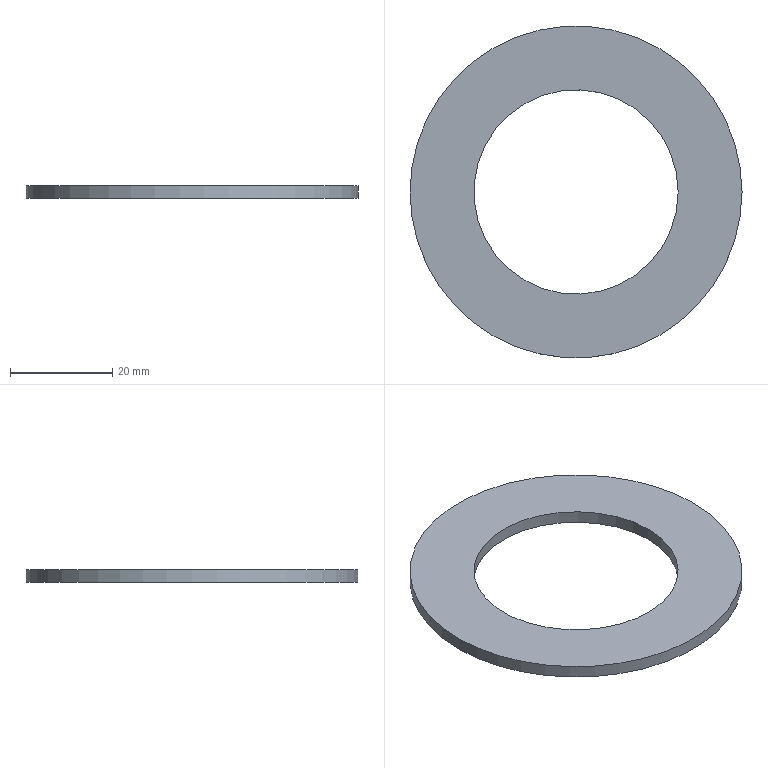Component | NX | WASHER_2 | 1 solid | 4 faces | box 65 x 65 x 2.5 mm | volume 5154 mm3 | cylinder 2 | plane 2 | commonest cylinder face diameters 65 x1 40 x1
STEP:
#1=CARTESIAN_POINT('',(0.,0.,0.));
#2=DIRECTION('',(0.,0.,1.));
#3=DIRECTION('',(1.,0.,0.));
#4=AXIS2_PLACEMENT_3D('',#1,#2,#3);
#5=CARTESIAN_POINT('',(-27.5,-165.,262.5));
#6=VERTEX_POINT('',#5);
#7=CARTESIAN_POINT('',(-60.,-165.,262.5));
#8=DIRECTION('',(0.,0.,-1.));
#9=DIRECTION('',(1.,0.,0.));
#10=AXIS2_PLACEMENT_3D('',#7,#8,#9);
#11=CIRCLE('',#10,32.5);
#12=CARTESIAN_POINT('',(-60.,-165.,262.5));
#13=DIRECTION('',(0.,0.,-1.));
#14=DIRECTION('',(-1.,0.,0.));
#15=AXIS2_PLACEMENT_3D('',#12,#13,#14);
#16=CYLINDRICAL_SURFACE('',#15,32.5);
#17=CARTESIAN_POINT('',(3.142,0.));
#18=DIRECTION('',(1.,0.));
#19=VECTOR('',#18,1.);
#20=LINE('',#17,#19);
#21=(GEOMETRIC_REPRESENTATION_CONTEXT(2)PARAMETRIC_REPRESENTATION_CONTEXT()REPRESENTATION_CONTEXT('',''));
#22=DEFINITIONAL_REPRESENTATION('',(#20),#21);
#23=PCURVE('',#16,#22);
#24=CARTESIAN_POINT('',(-60.,-165.,262.5));
#25=DIRECTION('',(0.,0.,-1.));
#26=DIRECTION('',(-1.,0.,0.));
#27=AXIS2_PLACEMENT_3D('',#24,#25,#26);
#28=PLANE('',#27);
#29=CARTESIAN_POINT('',(0.,0.));
#30=DIRECTION('',(-1.,0.));
#31=AXIS2_PLACEMENT_2D('',#29,#30);
#32=CIRCLE('',#31,32.5);
#33=(GEOMETRIC_REPRESENTATION_CONTEXT(2)PARAMETRIC_REPRESENTATION_CONTEXT()REPRESENTATION_CONTEXT('',''));
#34=DEFINITIONAL_REPRESENTATION('',(#32),#33);
#35=PCURVE('',#28,#34);
#36=SURFACE_CURVE('',#11,(#23,#35),.PCURVE_S1.);
#37=EDGE_CURVE('',#6,#6,#36,.T.);
#38=ORIENTED_EDGE('',*,*,#37,.T.);
#39=CARTESIAN_POINT('',(-27.5,-165.,260.));
#40=VERTEX_POINT('',#39);
#41=CARTESIAN_POINT('',(-27.5,-165.,262.5));
#42=CARTESIAN_POINT('',(-27.5,-165.,260.));
#43=B_SPLINE_CURVE_WITH_KNOTS('',1,(#41,#42),.UNSPECIFIED.,.F.,.F.,(2,2),(0.,2.5),.PIECEWISE_BEZIER_KNOTS.);
#44=CARTESIAN_POINT('',(9.425,0.));
#45=DIRECTION('',(0.,1.));
#46=VECTOR('',#45,1.);
#47=LINE('',#44,#46);
#48=(GEOMETRIC_REPRESENTATION_CONTEXT(2)PARAMETRIC_REPRESENTATION_CONTEXT()REPRESENTATION_CONTEXT('',''));
#49=DEFINITIONAL_REPRESENTATION('',(#47),#48);
#50=PCURVE('',#16,#49);
#51=CARTESIAN_POINT('',(3.142,0.));
#52=DIRECTION('',(0.,1.));
#53=VECTOR('',#52,1.);
#54=LINE('',#51,#53);
#55=(GEOMETRIC_REPRESENTATION_CONTEXT(2)PARAMETRIC_REPRESENTATION_CONTEXT()REPRESENTATION_CONTEXT('',''));
#56=DEFINITIONAL_REPRESENTATION('',(#54),#55);
#57=PCURVE('',#16,#56);
#58=SEAM_CURVE('',#43,(#50,#57),.PCURVE_S1.);
#59=EDGE_CURVE('',#6,#40,#58,.T.);
#60=ORIENTED_EDGE('',*,*,#59,.T.);
#61=CARTESIAN_POINT('',(-60.,-165.,260.));
#62=DIRECTION('',(0.,0.,-1.));
#63=DIRECTION('',(1.,0.,0.));
#64=AXIS2_PLACEMENT_3D('',#61,#62,#63);
#65=CIRCLE('',#64,32.5);
#66=CARTESIAN_POINT('',(3.142,2.5));
#67=DIRECTION('',(1.,0.));
#68=VECTOR('',#67,1.);
#69=LINE('',#66,#68);
#70=(GEOMETRIC_REPRESENTATION_CONTEXT(2)PARAMETRIC_REPRESENTATION_CONTEXT()REPRESENTATION_CONTEXT('',''));
#71=DEFINITIONAL_REPRESENTATION('',(#69),#70);
#72=PCURVE('',#16,#71);
#73=CARTESIAN_POINT('',(-60.,-165.,260.));
#74=DIRECTION('',(0.,0.,-1.));
#75=DIRECTION('',(-1.,0.,0.));
#76=AXIS2_PLACEMENT_3D('',#73,#74,#75);
#77=PLANE('',#76);
#78=CARTESIAN_POINT('',(0.,0.));
#79=DIRECTION('',(-1.,0.));
#80=AXIS2_PLACEMENT_2D('',#78,#79);
#81=CIRCLE('',#80,32.5);
#82=(GEOMETRIC_REPRESENTATION_CONTEXT(2)PARAMETRIC_REPRESENTATION_CONTEXT()REPRESENTATION_CONTEXT('',''));
#83=DEFINITIONAL_REPRESENTATION('',(#81),#82);
#84=PCURVE('',#77,#83);
#85=SURFACE_CURVE('',#65,(#72,#84),.PCURVE_S1.);
#86=EDGE_CURVE('',#40,#40,#85,.T.);
#87=ORIENTED_EDGE('',*,*,#86,.F.);
#88=ORIENTED_EDGE('',*,*,#59,.F.);
#89=EDGE_LOOP('',(#38,#60,#87,#88));
#90=FACE_BOUND('',#89,.T.);
#91=ADVANCED_FACE('',(#90),#16,.T.);
#92=CARTESIAN_POINT('',(-40.,-165.,262.5));
#93=VERTEX_POINT('',#92);
#94=CARTESIAN_POINT('',(-60.,-165.,262.5));
#95=DIRECTION('',(0.,0.,-1.));
#96=DIRECTION('',(1.,0.,0.));
#97=AXIS2_PLACEMENT_3D('',#94,#95,#96);
#98=CIRCLE('',#97,20.);
#99=CARTESIAN_POINT('',(-60.,-165.,262.5));
#100=DIRECTION('',(0.,0.,-1.));
#101=DIRECTION('',(-1.,0.,0.));
#102=AXIS2_PLACEMENT_3D('',#99,#100,#101);
#103=CYLINDRICAL_SURFACE('',#102,20.);
#104=CARTESIAN_POINT('',(3.142,0.));
#105=DIRECTION('',(1.,0.));
#106=VECTOR('',#105,1.);
#107=LINE('',#104,#106);
#108=(GEOMETRIC_REPRESENTATION_CONTEXT(2)PARAMETRIC_REPRESENTATION_CONTEXT()REPRESENTATION_CONTEXT('',''));
#109=DEFINITIONAL_REPRESENTATION('',(#107),#108);
#110=PCURVE('',#103,#109);
#111=CARTESIAN_POINT('',(0.,0.));
#112=DIRECTION('',(-1.,0.));
#113=AXIS2_PLACEMENT_2D('',#111,#112);
#114=CIRCLE('',#113,20.);
#115=(GEOMETRIC_REPRESENTATION_CONTEXT(2)PARAMETRIC_REPRESENTATION_CONTEXT()REPRESENTATION_CONTEXT('',''));
#116=DEFINITIONAL_REPRESENTATION('',(#114),#115);
#117=PCURVE('',#28,#116);
#118=SURFACE_CURVE('',#98,(#110,#117),.PCURVE_S1.);
#119=EDGE_CURVE('',#93,#93,#118,.T.);
#120=ORIENTED_EDGE('',*,*,#119,.T.);
#121=CARTESIAN_POINT('',(-40.,-165.,260.));
#122=VERTEX_POINT('',#121);
#123=CARTESIAN_POINT('',(-40.,-165.,262.5));
#124=CARTESIAN_POINT('',(-40.,-165.,260.));
#125=B_SPLINE_CURVE_WITH_KNOTS('',1,(#123,#124),.UNSPECIFIED.,.F.,.F.,(2,2),(0.,2.5),.PIECEWISE_BEZIER_KNOTS.);
#126=CARTESIAN_POINT('',(9.425,0.));
#127=DIRECTION('',(0.,1.));
#128=VECTOR('',#127,1.);
#129=LINE('',#126,#128);
#130=(GEOMETRIC_REPRESENTATION_CONTEXT(2)PARAMETRIC_REPRESENTATION_CONTEXT()REPRESENTATION_CONTEXT('',''));
#131=DEFINITIONAL_REPRESENTATION('',(#129),#130);
#132=PCURVE('',#103,#131);
#133=CARTESIAN_POINT('',(3.142,0.));
#134=DIRECTION('',(0.,1.));
#135=VECTOR('',#134,1.);
#136=LINE('',#133,#135);
#137=(GEOMETRIC_REPRESENTATION_CONTEXT(2)PARAMETRIC_REPRESENTATION_CONTEXT()REPRESENTATION_CONTEXT('',''));
#138=DEFINITIONAL_REPRESENTATION('',(#136),#137);
#139=PCURVE('',#103,#138);
#140=SEAM_CURVE('',#125,(#132,#139),.PCURVE_S1.);
#141=EDGE_CURVE('',#93,#122,#140,.T.);
#142=ORIENTED_EDGE('',*,*,#141,.T.);
#143=CARTESIAN_POINT('',(-60.,-165.,260.));
#144=DIRECTION('',(0.,0.,-1.));
#145=DIRECTION('',(1.,0.,0.));
#146=AXIS2_PLACEMENT_3D('',#143,#144,#145);
#147=CIRCLE('',#146,20.);
#148=CARTESIAN_POINT('',(3.142,2.5));
#149=DIRECTION('',(1.,0.));
#150=VECTOR('',#149,1.);
#151=LINE('',#148,#150);
#152=(GEOMETRIC_REPRESENTATION_CONTEXT(2)PARAMETRIC_REPRESENTATION_CONTEXT()REPRESENTATION_CONTEXT('',''));
#153=DEFINITIONAL_REPRESENTATION('',(#151),#152);
#154=PCURVE('',#103,#153);
#155=CARTESIAN_POINT('',(0.,0.));
#156=DIRECTION('',(-1.,0.));
#157=AXIS2_PLACEMENT_2D('',#155,#156);
#158=CIRCLE('',#157,20.);
#159=(GEOMETRIC_REPRESENTATION_CONTEXT(2)PARAMETRIC_REPRESENTATION_CONTEXT()REPRESENTATION_CONTEXT('',''));
#160=DEFINITIONAL_REPRESENTATION('',(#158),#159);
#161=PCURVE('',#77,#160);
#162=SURFACE_CURVE('',#147,(#154,#161),.PCURVE_S1.);
#163=EDGE_CURVE('',#122,#122,#162,.T.);
#164=ORIENTED_EDGE('',*,*,#163,.F.);
#165=ORIENTED_EDGE('',*,*,#141,.F.);
#166=EDGE_LOOP('',(#120,#142,#164,#165));
#167=FACE_BOUND('',#166,.F.);
#168=ADVANCED_FACE('',(#167),#103,.F.);
#169=ORIENTED_EDGE('',*,*,#37,.F.);
#170=EDGE_LOOP('',(#169));
#171=FACE_BOUND('',#170,.T.);
#172=ORIENTED_EDGE('',*,*,#119,.T.);
#173=EDGE_LOOP('',(#172));
#174=FACE_BOUND('',#173,.T.);
#175=ADVANCED_FACE('',(#171,#174),#28,.F.);
#176=ORIENTED_EDGE('',*,*,#86,.T.);
#177=EDGE_LOOP('',(#176));
#178=FACE_BOUND('',#177,.T.);
#179=ORIENTED_EDGE('',*,*,#163,.F.);
#180=EDGE_LOOP('',(#179));
#181=FACE_BOUND('',#180,.T.);
#182=ADVANCED_FACE('',(#178,#181),#77,.T.);
#183=CLOSED_SHELL('',(#91,#168,#175,#182));
#184=MANIFOLD_SOLID_BREP('',#183);
#185=(LENGTH_UNIT()NAMED_UNIT(*)SI_UNIT(.MILLI.,.METRE.));
#186=UNCERTAINTY_MEASURE_WITH_UNIT(LENGTH_MEASURE(0.00001),#185,'','');
#187=(NAMED_UNIT(*)PLANE_ANGLE_UNIT()SI_UNIT($,.RADIAN.));
#188=(NAMED_UNIT(*)SI_UNIT($,.STERADIAN.)SOLID_ANGLE_UNIT());
#189=(GEOMETRIC_REPRESENTATION_CONTEXT(3)GLOBAL_UNCERTAINTY_ASSIGNED_CONTEXT((#186))GLOBAL_UNIT_ASSIGNED_CONTEXT((#185,#187,#188))REPRESENTATION_CONTEXT('',''));
#190=ADVANCED_BREP_SHAPE_REPRESENTATION('',(#4,#184),#189);